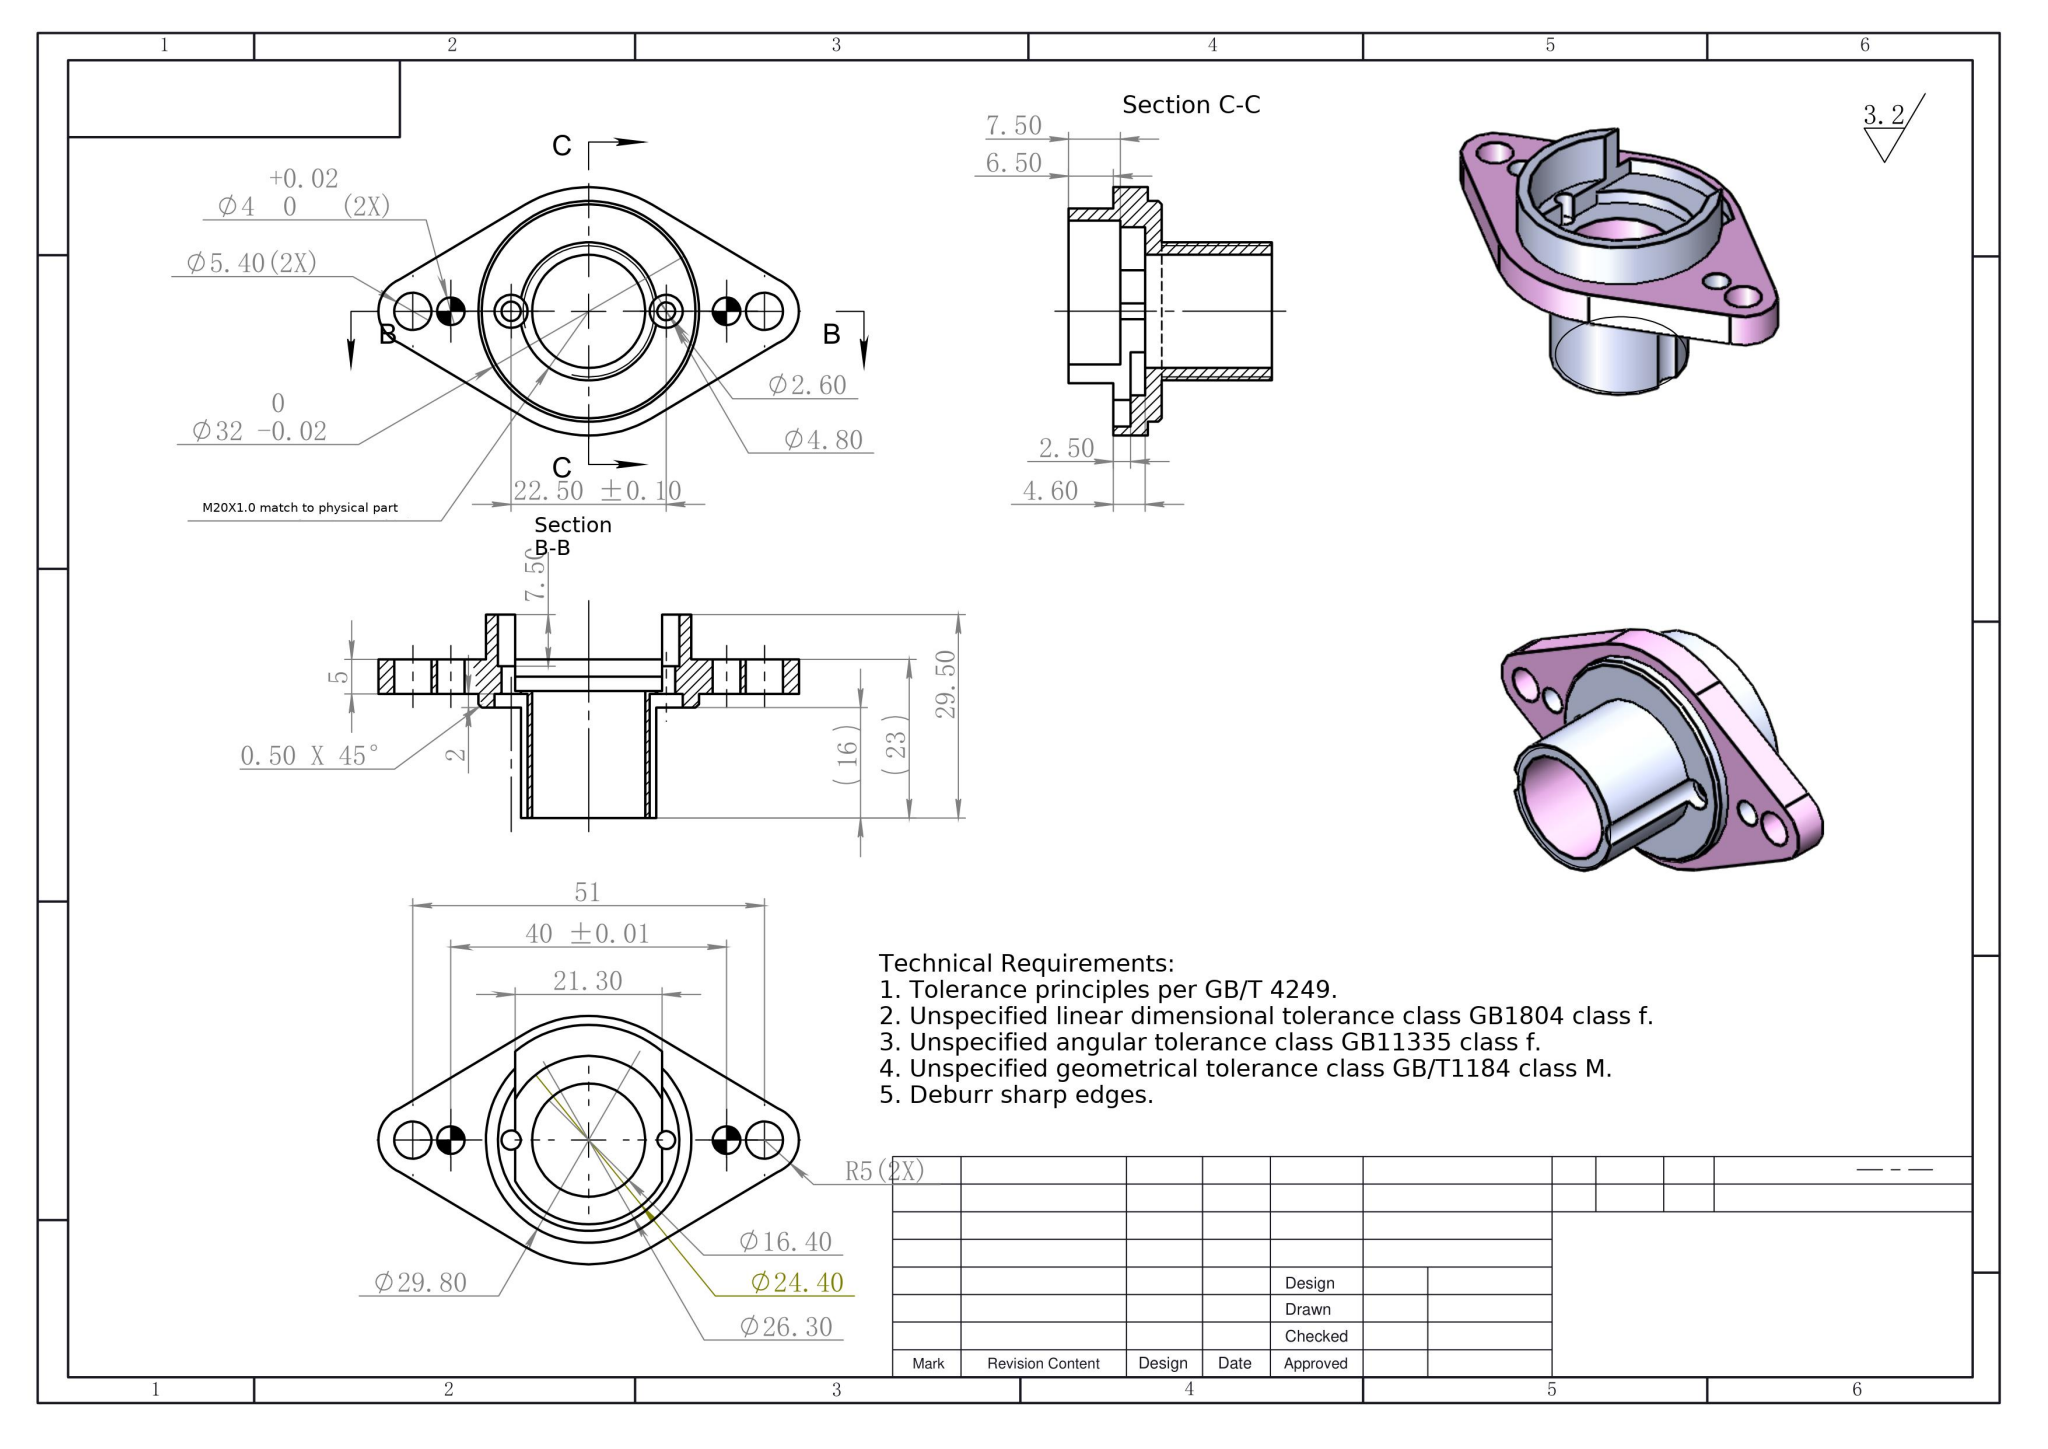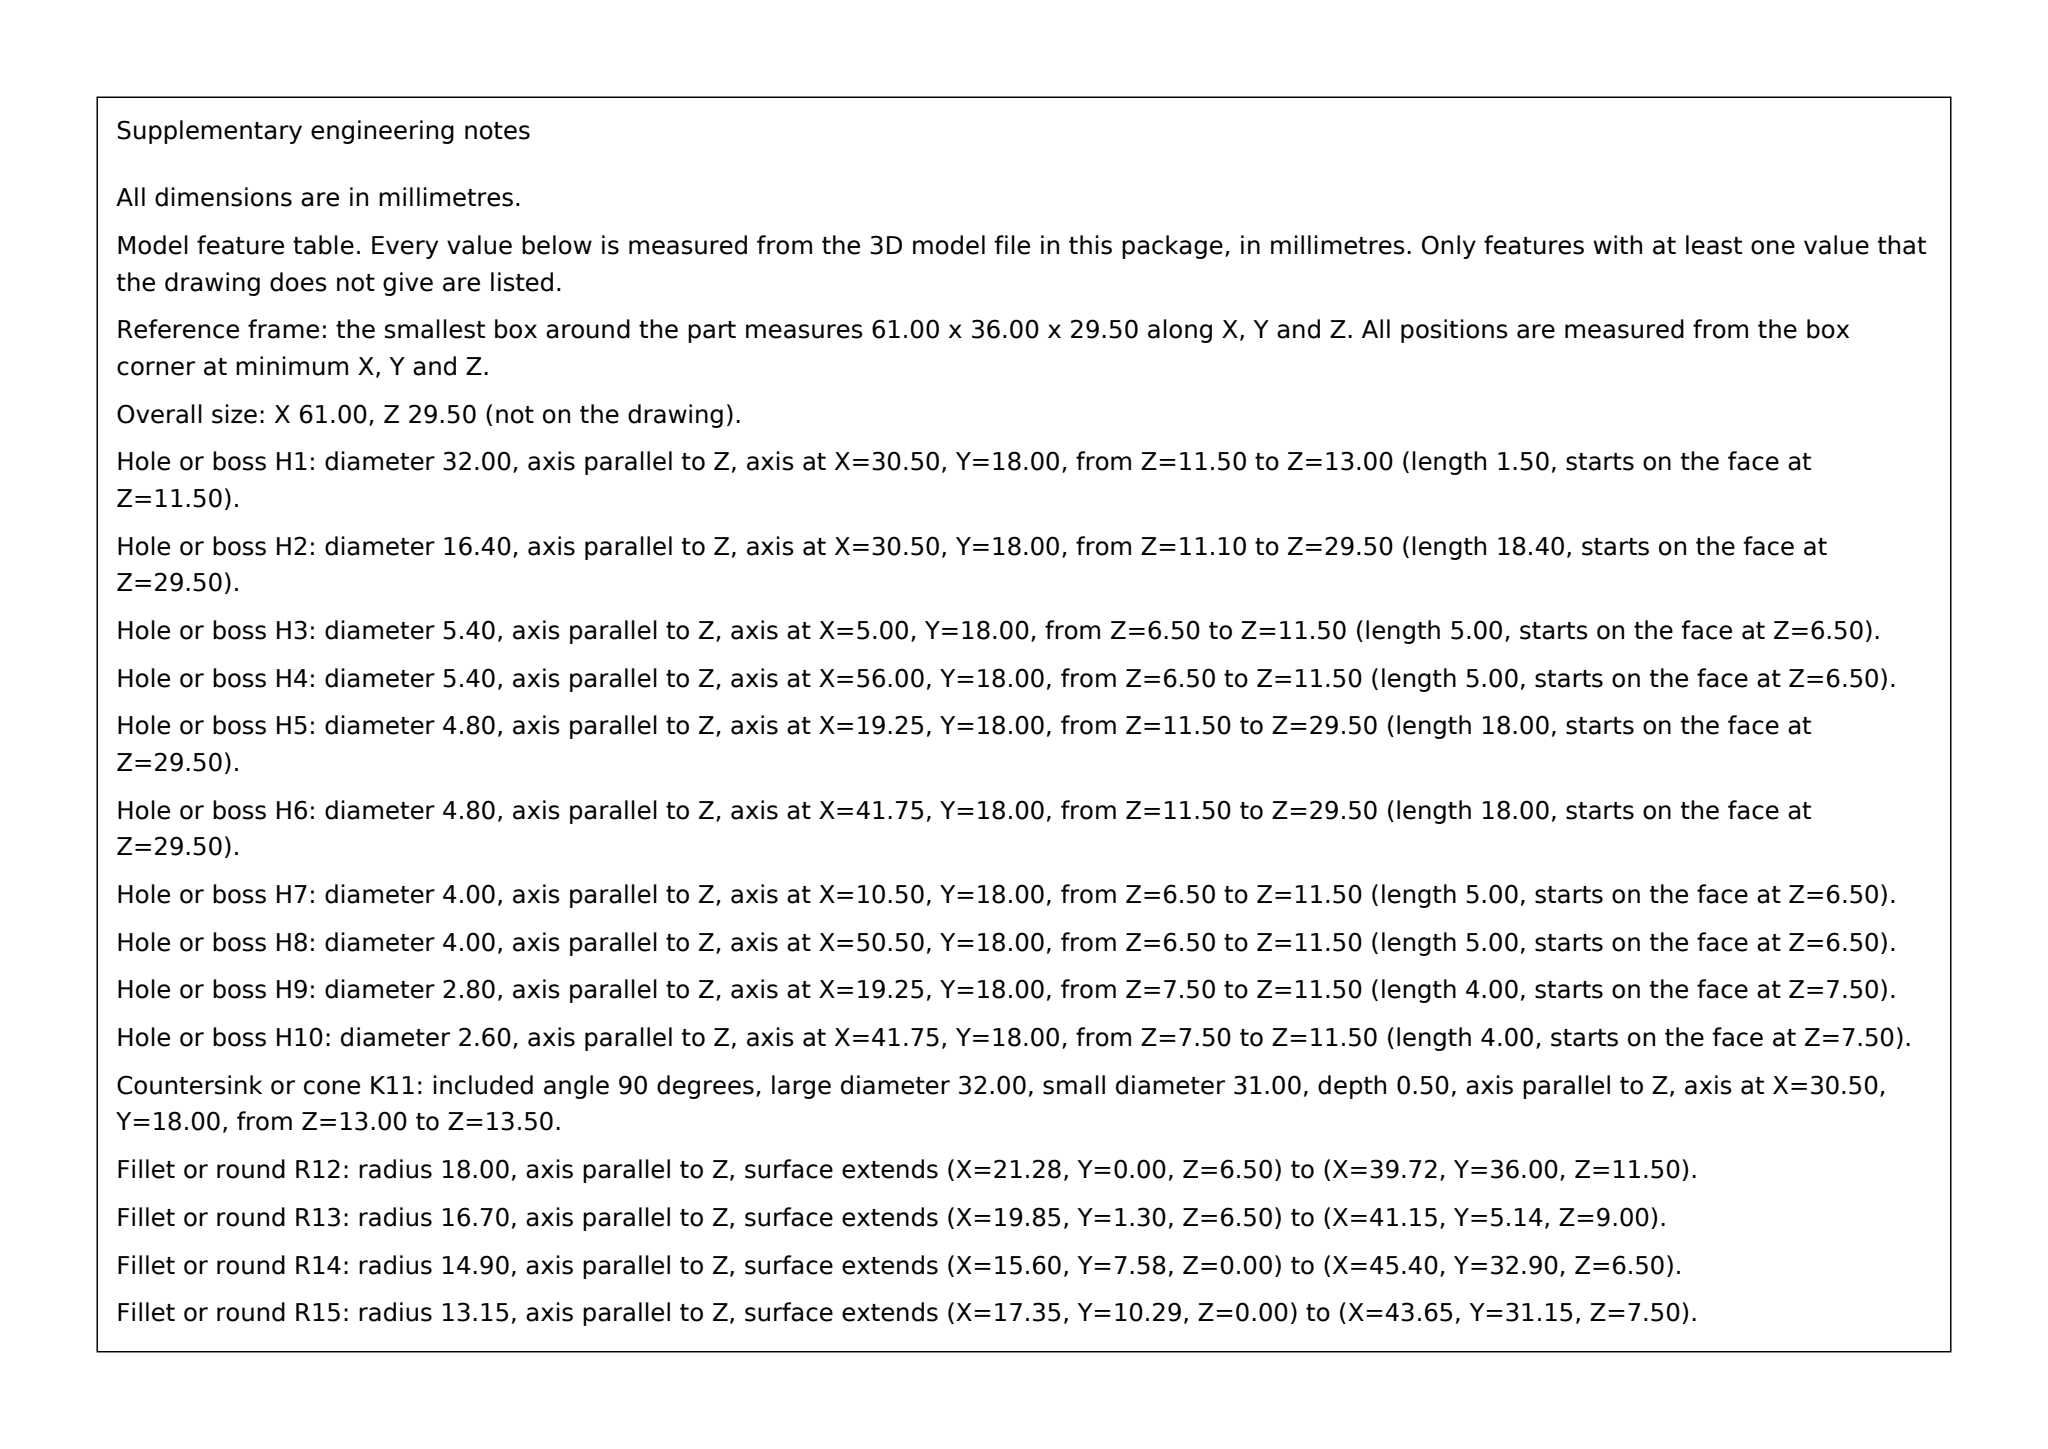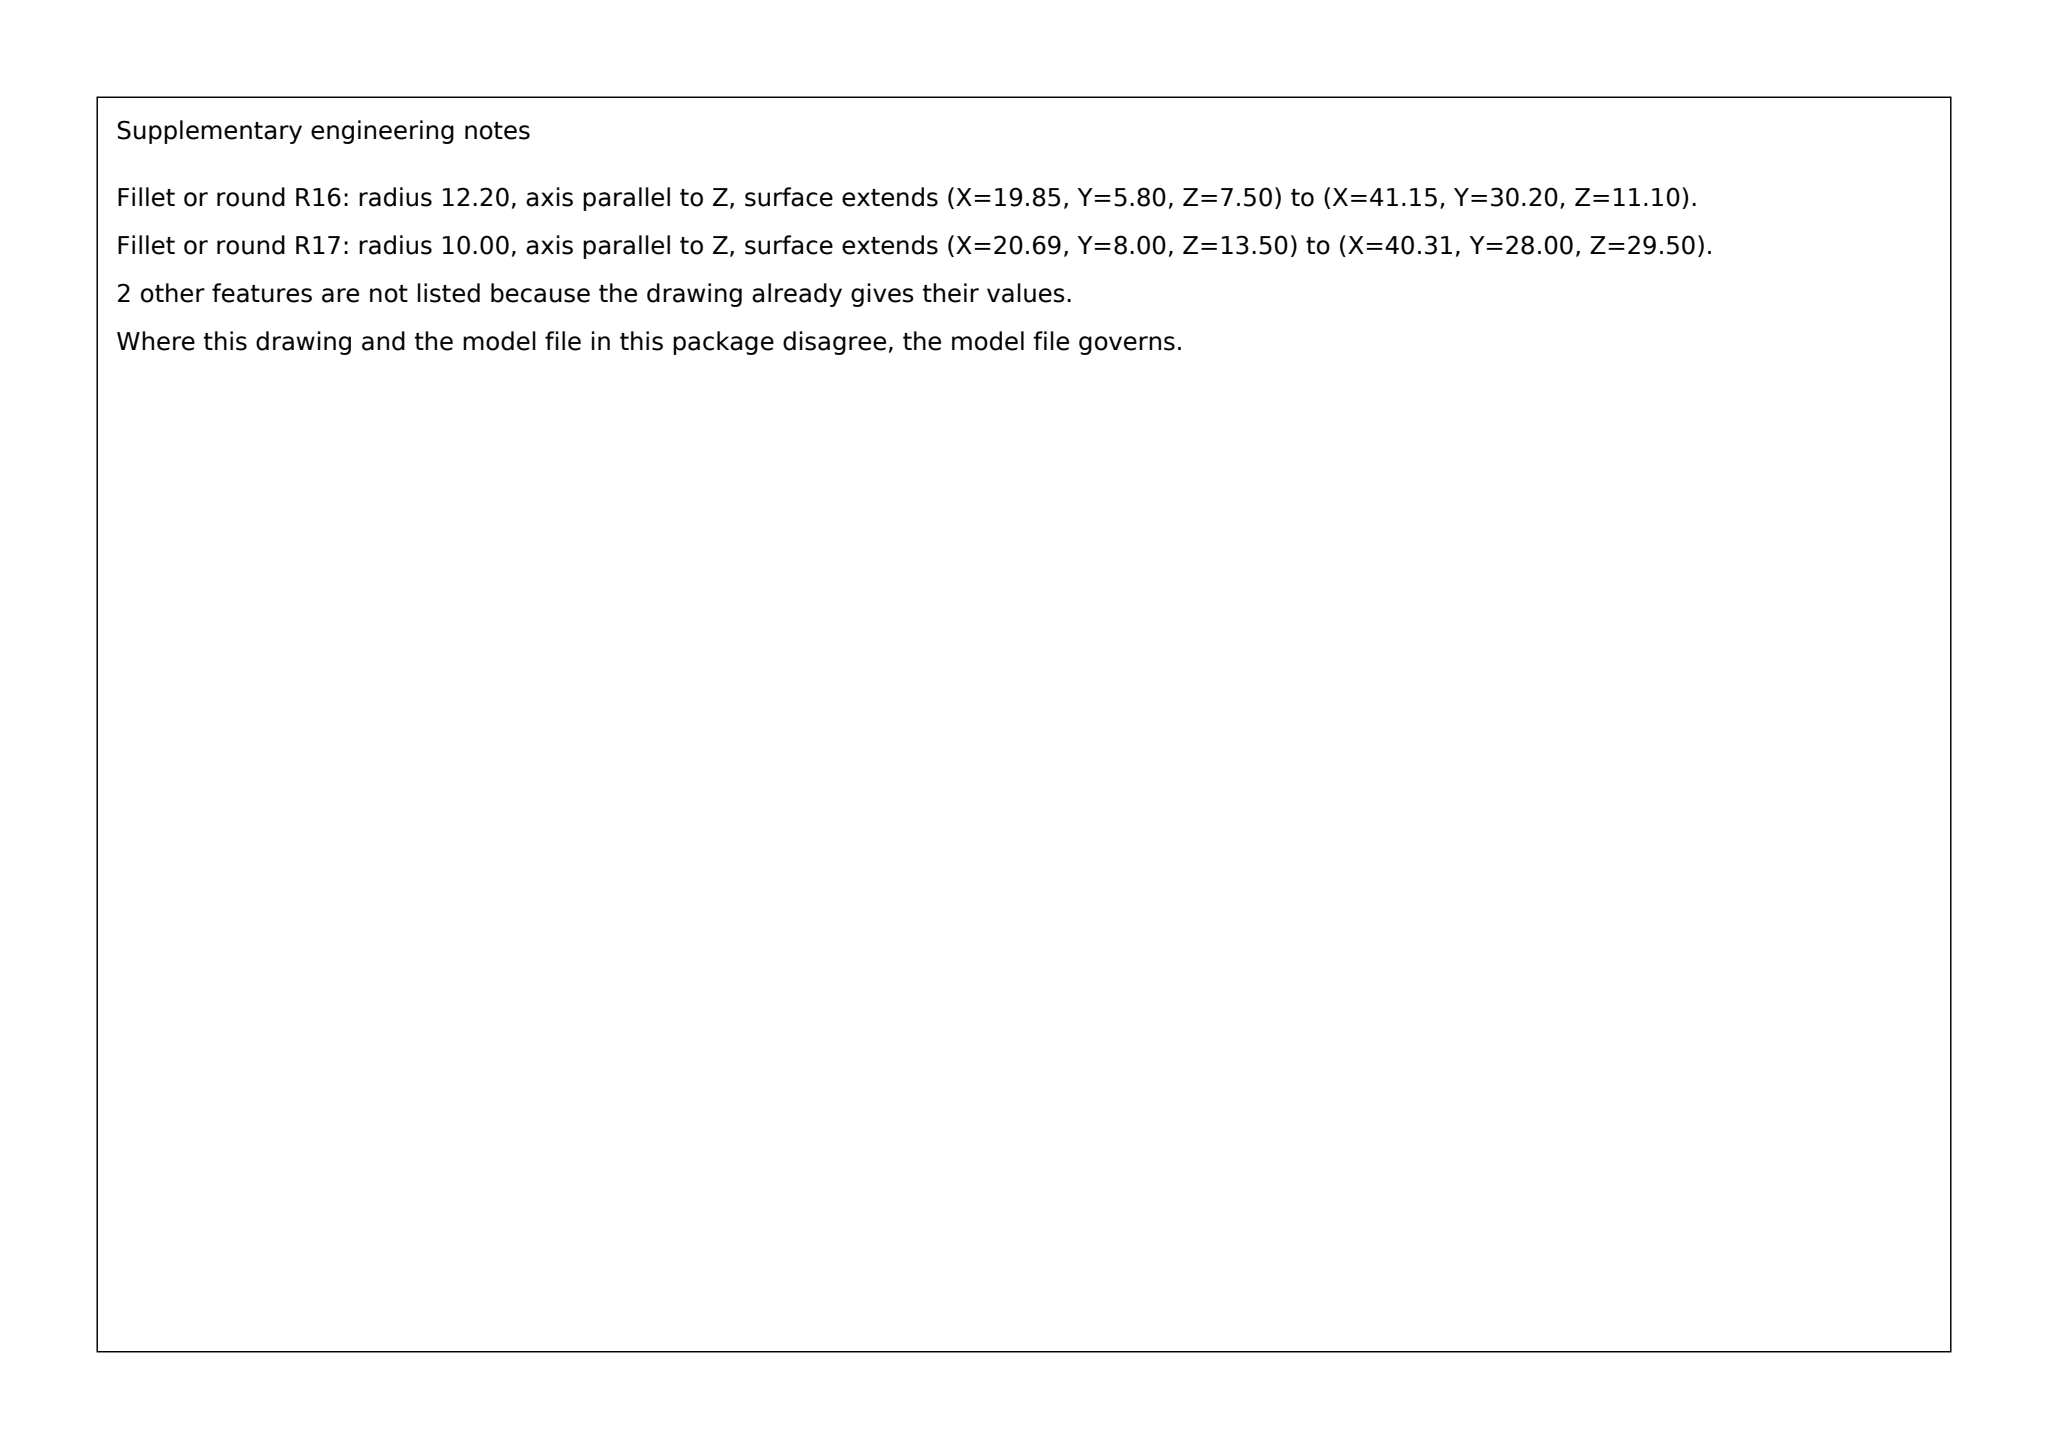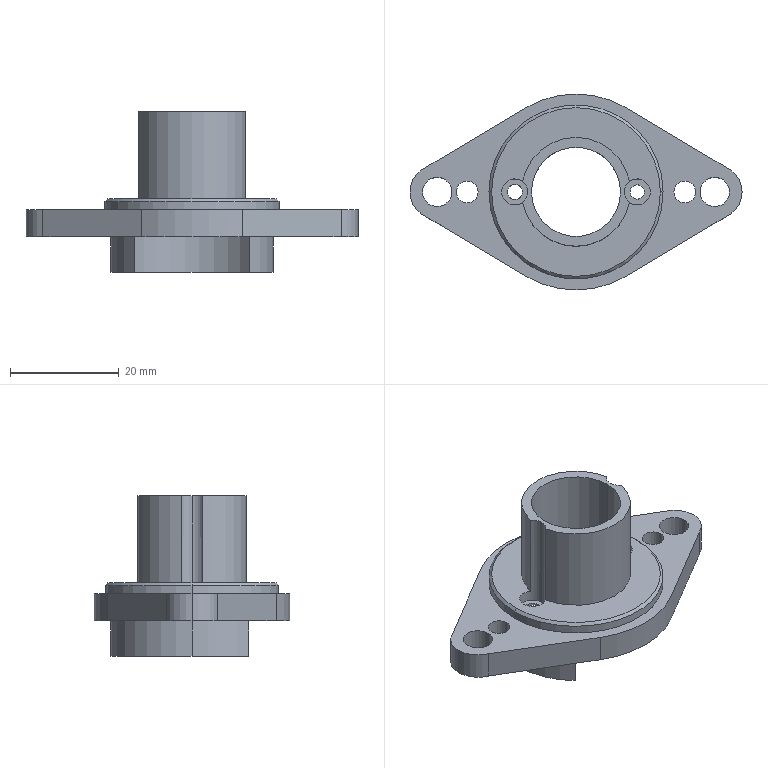Part | SolidWorks | mm | 1 solid | 56 faces | box 61 x 36 x 29.5 mm | volume 7543 mm3 | cylinder 36 | plane 18 | cone 2 | commonest cylinder face diameters 4 x4 4.8 x4 5.4 x4 26.3 x3 29.8 x3 10 x3 32 x2 16.4 x2
build123d program:
from build123d import *

# Parameters (mm, degrees)
SKETCH1_R                    = 8.2
SKETCH1_R_2                  = 2.7
EXTRUDE1_DEPTH               = 2.5
SKETCH2_R                    = 16
SKETCH2_R_2                  = 8.2
EXTRUDE2_DEPTH               = 2
SKETCH3_R                    = 10
SKETCH3_R_2                  = 8.2
EXTRUDE3_DEPTH               = 16
SKETCH4_R                    = 2.4
EXTRUDE4_DEPTH               = 18
EXTRUDE5_START               = 6.5
SKETCH6_R                    = 14.9
SKETCH6_R_2                  = 8.2
EXTRUDE5_DEPTH               = 6.5
SKETCH7_R                    = 13.15
EXTRUDE6_DEPTH               = 6.5
EXTRUDE7_DEPTH               = 9
SKETCH9_R                    = 1.4
SKETCH9_R_2                  = 1.3
EXTRUDE8_DEPTH               = 9
EXTRUDE9_DEPTH               = 4.6
F_4_0_4_DIAMETER_HOLE1_D     = 4
F_4_0_4_DIAMETER_HOLE1_DEPTH = 20
F_4_0_4_DIAMETER_HOLE1_TIP   = 1.202
SKETCH15_R                   = 13.15
CUT_EXTRUDE2_DEPTH           = 1
CHAMFER1_SIZE                = 0.5


with BuildPart() as part:
    # Sketch1 → Extrude1 (new, symmetric)
    with BuildSketch(Plane.XY):
        with BuildLine():
            Line((-27.389, 4.63), (-9.216, 15.462))
            ThreePointArc((-9.216, 15.462), (0, 18), (9.216, 15.462))
            Line((9.216, 15.462), (27.389, 4.63))
            ThreePointArc((27.389, 4.63), (30.5, 0), (27.389, -4.63))
            Line((27.389, -4.63), (9.216, -15.462))
            ThreePointArc((9.216, -15.462), (0, -18), (-9.216, -15.462))
            Line((-9.216, -15.462), (-27.389, -4.63))
            ThreePointArc((-27.389, -4.63), (-30.5, 0), (-27.389, 4.63))
        make_face()
        Circle(SKETCH1_R, mode=Mode.SUBTRACT)
        with Locations((-25.5, 0)):
            Circle(SKETCH1_R_2, mode=Mode.SUBTRACT)
        with Locations((25.5, 0)):
            Circle(SKETCH1_R_2, mode=Mode.SUBTRACT)
    extrude(amount=EXTRUDE1_DEPTH, both=True)

    # Sketch2 → Extrude2 (add)
    with BuildSketch(Plane.XY.offset(2.5)):
        Circle(SKETCH2_R)
        Circle(SKETCH2_R_2, mode=Mode.SUBTRACT)
    extrude(amount=EXTRUDE2_DEPTH)

    # Sketch3 → Extrude3 (add)
    with BuildSketch(Plane.XY.offset(4.5)):
        Circle(SKETCH3_R)
        Circle(SKETCH3_R_2, mode=Mode.SUBTRACT)
    extrude(amount=EXTRUDE3_DEPTH)

    # Sketch4 → Extrude4 (cut)
    with BuildSketch(Plane.XY.offset(20.5)):
        with Locations((-11.25, 0)):
            Circle(SKETCH4_R)
        with Locations((11.25, 0)):
            Circle(SKETCH4_R)
    extrude(amount=-EXTRUDE4_DEPTH, mode=Mode.SUBTRACT)

    # Sketch6 → Extrude5 (add)
    with BuildSketch(Plane(origin=(0, 0, -2.5), x_dir=(-1, 0, 0), z_dir=(0, 0, -1)).offset(EXTRUDE5_START)):
        with Locations(Location((0, 0, 0), (0, 0, 180))):
            Circle(SKETCH6_R)
        Circle(SKETCH6_R_2, mode=Mode.SUBTRACT)
    extrude(amount=-EXTRUDE5_DEPTH)

    # Sketch7 → Extrude6 (cut)
    with BuildSketch(Plane(origin=(0, 0, -9), x_dir=(-1, 0, 0), z_dir=(0, 0, -1))):
        Circle(SKETCH7_R)
    extrude(amount=-EXTRUDE6_DEPTH, mode=Mode.SUBTRACT)

    # Sketch8 → Extrude7 (cut)
    with BuildSketch(Plane(origin=(0, 0, -9), x_dir=(-1, 0, 0), z_dir=(0, 0, -1))):
        with BuildLine():
            Line((-10.65, 5.951), (-10.65, -12.863))
            ThreePointArc((-10.65, -12.863), (0, -16.7), (10.65, -12.863))
            Line((10.65, -12.863), (10.65, 5.951))
            ThreePointArc((10.65, 5.951), (0, 12.2), (-10.65, 5.951))
        make_face()
    extrude(amount=-EXTRUDE7_DEPTH, mode=Mode.SUBTRACT)

    # Sketch9 → Extrude8 (cut)
    with BuildSketch(Plane.XY.offset(4.5)):
        with Locations((-11.25, 0)):
            Circle(SKETCH9_R)
        with Locations((11.25, 0)):
            Circle(SKETCH9_R_2)
    extrude(amount=-EXTRUDE8_DEPTH, mode=Mode.SUBTRACT)

    # Sketch10 → Extrude9 (cut)
    with BuildSketch(Plane(origin=(0, 0, -2.5), x_dir=(-1, 0, 0), z_dir=(0, 0, -1))):
        with BuildLine():
            Line((-10.65, -5.951), (-10.65, 5.951))
            ThreePointArc((-10.65, 5.951), (0, 12.2), (10.65, 5.951))
            Line((10.65, 5.951), (10.65, -5.951))
            ThreePointArc((10.65, -5.951), (0, -12.2), (-10.65, -5.951))
        make_face()
    extrude(amount=-EXTRUDE9_DEPTH, mode=Mode.SUBTRACT)

    # 4.0 _4_ Diameter Hole1
    with Locations(Plane(origin=(0, 0, -2.5), x_dir=(-1, 0, 0), z_dir=(0, 0, -1))):
        with Locations((-20, 0), (20, 0)):
            Hole(F_4_0_4_DIAMETER_HOLE1_D / 2, depth=F_4_0_4_DIAMETER_HOLE1_DEPTH)
            with Locations((0, 0, -(F_4_0_4_DIAMETER_HOLE1_DEPTH + F_4_0_4_DIAMETER_HOLE1_TIP / 2))):  # 118° drill point
                Cone(0, F_4_0_4_DIAMETER_HOLE1_D / 2, F_4_0_4_DIAMETER_HOLE1_TIP, mode=Mode.SUBTRACT)

    # Sketch15 → Cut-Extrude2 (cut)
    with BuildSketch(Plane(origin=(0, 0, -2.5), x_dir=(-1, 0, 0), z_dir=(0, 0, -1))):
        Circle(SKETCH15_R)
    extrude(amount=-CUT_EXTRUDE2_DEPTH, mode=Mode.SUBTRACT)

    # Chamfer1
    chamfer1_edges = [part.edges().sort_by_distance(p)[0] for p in [
        (-16, 0, 4.5),
    ]]
    chamfer(chamfer1_edges, length=CHAMFER1_SIZE)


solid = part.part